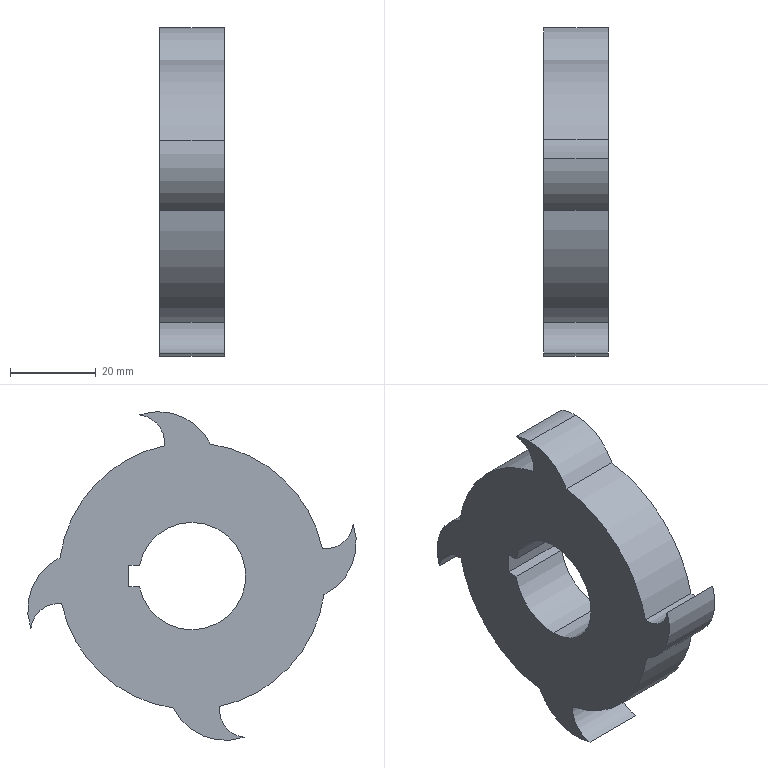Component | SolidWorks | CrushingCutterDisc-1 | 1 solid | 22 faces | box 15 x 76.47 x 76.47 mm | volume 41680 mm3 | cylinder 17 | plane 5 | commonest cylinder face diameters 12.958 x5 26.806 x5 62 x4 25 x3
build123d program:
from build123d import *

# Parameters (mm, degrees)
BOSS_EXTRUDE1_DEPTH = 15
CUT_EXTRUDE1_DEPTH  = 15


with BuildPart() as part:
    # Sketch1 → Boss-Extrude1 (new body)
    with BuildSketch(Plane.XY):
        with BuildLine():
            ThreePointArc((-30.696, -4.328), (-22.657, -21.158), (-6.415, -30.329))
            ThreePointArc((-6.415, -30.329), (-7.787, -35.094), (-12.127, -37.494))
            ThreePointArc((-12.127, -37.494), (-2.607, -37.222), (4.328, -30.696))
            ThreePointArc((4.328, -30.696), (21.158, -22.657), (30.329, -6.415))
            ThreePointArc((30.329, -6.415), (35.094, -7.787), (37.494, -12.127))
            ThreePointArc((37.494, -12.127), (37.222, -2.607), (30.696, 4.328))
            ThreePointArc((30.696, 4.328), (22.657, 21.158), (6.415, 30.329))
            ThreePointArc((6.415, 30.329), (7.787, 35.094), (12.127, 37.494))
            ThreePointArc((12.127, 37.494), (2.607, 37.222), (-4.328, 30.696))
            ThreePointArc((-4.328, 30.696), (-21.158, 22.657), (-30.329, 6.415))
            ThreePointArc((-30.329, 6.415), (-35.094, 7.787), (-37.494, 12.127))
            ThreePointArc((-37.494, 12.127), (-37.222, 2.607), (-30.696, -4.328))
        make_face()
    extrude(amount=BOSS_EXTRUDE1_DEPTH)

    # Sketch2 → Cut-Extrude1 (cut)
    with BuildSketch(Plane.XY.offset(15)):
        with BuildLine():
            Line((-2.499, 12.248), (-2.499, 14.709))
            Line((-2.499, 14.709), (2.501, 14.709))
            Line((2.501, 14.709), (2.501, 12.247))
            ThreePointArc((2.501, 12.247), (-0.001021, -12.5), (-2.499, 12.248))
        make_face()
    extrude(amount=-CUT_EXTRUDE1_DEPTH, mode=Mode.SUBTRACT)


solid = part.part

# Placed as in the assembly
solid = solid.moved(Location((386.19, 335.1, -35), (0, 90, 0)))
STEP:
#1=COLOUR_RGB('',0.7922,0.8196,0.9333);
#2=FILL_AREA_STYLE_COLOUR('',#1);
#3=FILL_AREA_STYLE('',(#2));
#4=SURFACE_STYLE_FILL_AREA(#3);
#5=SURFACE_SIDE_STYLE('',(#4));
#6=SURFACE_STYLE_USAGE(.BOTH.,#5);
#7=PRESENTATION_STYLE_ASSIGNMENT((#6));
#8=CARTESIAN_POINT('',(15.204,13.193,-0.8858));
#9=VERTEX_POINT('',#8);
#10=CARTESIAN_POINT('',(15.204,13.193,-1.87));
#11=VERTEX_POINT('',#10);
#12=CARTESIAN_POINT('',(15.204,13.193,-1.378));
#13=DIRECTION('',(1.,0.,-0.));
#14=DIRECTION('',(0.,0.,-1.));
#15=AXIS2_PLACEMENT_3D('',#12,#13,#14);
#16=CIRCLE('',#15,0.4921);
#17=EDGE_CURVE('',#9,#11,#16,.T.);
#18=ORIENTED_EDGE('',*,*,#17,.F.);
#19=CARTESIAN_POINT('',(15.795,13.193,-0.8858));
#20=VERTEX_POINT('',#19);
#21=CARTESIAN_POINT('',(15.204,13.193,-0.8858));
#22=DIRECTION('',(1.,0.,-0.));
#23=VECTOR('',#22,39.37);
#24=LINE('',#21,#23);
#25=EDGE_CURVE('',#9,#20,#24,.T.);
#26=ORIENTED_EDGE('',*,*,#25,.T.);
#27=CARTESIAN_POINT('',(15.795,13.193,-1.87));
#28=VERTEX_POINT('',#27);
#29=CARTESIAN_POINT('',(15.795,13.193,-1.378));
#30=DIRECTION('',(1.,0.,-0.));
#31=DIRECTION('',(0.,0.,-1.));
#32=AXIS2_PLACEMENT_3D('',#29,#30,#31);
#33=CIRCLE('',#32,0.4921);
#34=EDGE_CURVE('',#20,#28,#33,.T.);
#35=ORIENTED_EDGE('',*,*,#34,.T.);
#36=CARTESIAN_POINT('',(15.204,13.193,-1.87));
#37=DIRECTION('',(1.,0.,-0.));
#38=VECTOR('',#37,39.37);
#39=LINE('',#36,#38);
#40=EDGE_CURVE('',#11,#28,#39,.T.);
#41=ORIENTED_EDGE('',*,*,#40,.F.);
#42=EDGE_LOOP('',(#18,#26,#35,#41));
#43=FACE_OUTER_BOUND('',#42,.T.);
#44=CARTESIAN_POINT('',(15.204,13.193,-1.378));
#45=DIRECTION('',(1.,0.,-0.));
#46=DIRECTION('',(0.,0.,-1.));
#47=AXIS2_PLACEMENT_3D('',#44,#45,#46);
#48=CYLINDRICAL_SURFACE('',#47,0.4921);
#49=ADVANCED_FACE('',(#43),#48,.F.);
#50=CARTESIAN_POINT('',(15.204,13.675,-1.476));
#51=VERTEX_POINT('',#50);
#52=CARTESIAN_POINT('',(15.204,13.193,-1.378));
#53=DIRECTION('',(1.,0.,-0.));
#54=DIRECTION('',(0.,0.,-1.));
#55=AXIS2_PLACEMENT_3D('',#52,#53,#54);
#56=CIRCLE('',#55,0.4921);
#57=EDGE_CURVE('',#11,#51,#56,.T.);
#58=ORIENTED_EDGE('',*,*,#57,.F.);
#59=ORIENTED_EDGE('',*,*,#40,.T.);
#60=CARTESIAN_POINT('',(15.795,13.675,-1.476));
#61=VERTEX_POINT('',#60);
#62=CARTESIAN_POINT('',(15.795,13.193,-1.378));
#63=DIRECTION('',(1.,0.,-0.));
#64=DIRECTION('',(0.,0.,-1.));
#65=AXIS2_PLACEMENT_3D('',#62,#63,#64);
#66=CIRCLE('',#65,0.4921);
#67=EDGE_CURVE('',#28,#61,#66,.T.);
#68=ORIENTED_EDGE('',*,*,#67,.T.);
#69=CARTESIAN_POINT('',(15.204,13.675,-1.476));
#70=DIRECTION('',(1.,0.,-0.));
#71=VECTOR('',#70,39.37);
#72=LINE('',#69,#71);
#73=EDGE_CURVE('',#51,#61,#72,.T.);
#74=ORIENTED_EDGE('',*,*,#73,.F.);
#75=EDGE_LOOP('',(#58,#59,#68,#74));
#76=FACE_OUTER_BOUND('',#75,.T.);
#77=CARTESIAN_POINT('',(15.204,13.193,-1.378));
#78=DIRECTION('',(1.,0.,-0.));
#79=DIRECTION('',(0.,0.,-1.));
#80=AXIS2_PLACEMENT_3D('',#77,#78,#79);
#81=CYLINDRICAL_SURFACE('',#80,0.4921);
#82=ADVANCED_FACE('',(#76),#81,.F.);
#83=CARTESIAN_POINT('',(15.795,14.416,-1.629));
#84=VERTEX_POINT('',#83);
#85=CARTESIAN_POINT('',(15.795,14.669,-1.855));
#86=VERTEX_POINT('',#85);
#87=CARTESIAN_POINT('',(15.795,14.416,-1.884));
#88=DIRECTION('',(-1.,-0.,0.));
#89=DIRECTION('',(0.,0.,1.));
#90=AXIS2_PLACEMENT_3D('',#87,#88,#89);
#91=CIRCLE('',#90,0.2551);
#92=EDGE_CURVE('',#84,#86,#91,.T.);
#93=ORIENTED_EDGE('',*,*,#92,.F.);
#94=CARTESIAN_POINT('',(15.204,14.416,-1.629));
#95=VERTEX_POINT('',#94);
#96=CARTESIAN_POINT('',(15.795,14.416,-1.629));
#97=DIRECTION('',(-1.,-0.,0.));
#98=VECTOR('',#97,39.37);
#99=LINE('',#96,#98);
#100=EDGE_CURVE('',#84,#95,#99,.T.);
#101=ORIENTED_EDGE('',*,*,#100,.T.);
#102=CARTESIAN_POINT('',(15.204,14.669,-1.855));
#103=VERTEX_POINT('',#102);
#104=CARTESIAN_POINT('',(15.204,14.416,-1.884));
#105=DIRECTION('',(-1.,-0.,0.));
#106=DIRECTION('',(0.,0.,1.));
#107=AXIS2_PLACEMENT_3D('',#104,#105,#106);
#108=CIRCLE('',#107,0.2551);
#109=EDGE_CURVE('',#95,#103,#108,.T.);
#110=ORIENTED_EDGE('',*,*,#109,.T.);
#111=CARTESIAN_POINT('',(15.795,14.669,-1.855));
#112=DIRECTION('',(-1.,-0.,0.));
#113=VECTOR('',#112,39.37);
#114=LINE('',#111,#113);
#115=EDGE_CURVE('',#86,#103,#114,.T.);
#116=ORIENTED_EDGE('',*,*,#115,.F.);
#117=EDGE_LOOP('',(#93,#101,#110,#116));
#118=FACE_OUTER_BOUND('',#117,.T.);
#119=CARTESIAN_POINT('',(15.795,14.416,-1.884));
#120=DIRECTION('',(-1.,-0.,0.));
#121=DIRECTION('',(0.,0.,1.));
#122=AXIS2_PLACEMENT_3D('',#119,#120,#121);
#123=CYLINDRICAL_SURFACE('',#122,0.2551);
#124=ADVANCED_FACE('',(#118),#123,.F.);
#125=CARTESIAN_POINT('',(15.795,13.497,0.1275));
#126=VERTEX_POINT('',#125);
#127=CARTESIAN_POINT('',(15.795,13.023,-0.1694));
#128=VERTEX_POINT('',#127);
#129=CARTESIAN_POINT('',(15.795,13.497,-0.4002));
#130=DIRECTION('',(1.,0.,-0.));
#131=DIRECTION('',(0.,0.,1.));
#132=AXIS2_PLACEMENT_3D('',#129,#130,#131);
#133=CIRCLE('',#132,0.5277);
#134=EDGE_CURVE('',#126,#128,#133,.T.);
#135=ORIENTED_EDGE('',*,*,#134,.F.);
#136=CARTESIAN_POINT('',(15.204,13.497,0.1275));
#137=VERTEX_POINT('',#136);
#138=CARTESIAN_POINT('',(15.795,13.497,0.1275));
#139=DIRECTION('',(-1.,-0.,0.));
#140=VECTOR('',#139,39.37);
#141=LINE('',#138,#140);
#142=EDGE_CURVE('',#126,#137,#141,.T.);
#143=ORIENTED_EDGE('',*,*,#142,.T.);
#144=CARTESIAN_POINT('',(15.204,13.023,-0.1694));
#145=VERTEX_POINT('',#144);
#146=CARTESIAN_POINT('',(15.204,13.497,-0.4002));
#147=DIRECTION('',(1.,0.,-0.));
#148=DIRECTION('',(0.,0.,1.));
#149=AXIS2_PLACEMENT_3D('',#146,#147,#148);
#150=CIRCLE('',#149,0.5277);
#151=EDGE_CURVE('',#137,#145,#150,.T.);
#152=ORIENTED_EDGE('',*,*,#151,.T.);
#153=CARTESIAN_POINT('',(15.795,13.023,-0.1694));
#154=DIRECTION('',(-1.,-0.,0.));
#155=VECTOR('',#154,39.37);
#156=LINE('',#153,#155);
#157=EDGE_CURVE('',#128,#145,#156,.T.);
#158=ORIENTED_EDGE('',*,*,#157,.F.);
#159=EDGE_LOOP('',(#135,#143,#152,#158));
#160=FACE_OUTER_BOUND('',#159,.T.);
#161=CARTESIAN_POINT('',(15.795,13.497,-0.4002));
#162=DIRECTION('',(-1.,-0.,0.));
#163=DIRECTION('',(0.,0.,1.));
#164=AXIS2_PLACEMENT_3D('',#161,#162,#163);
#165=CYLINDRICAL_SURFACE('',#164,0.5277);
#166=ADVANCED_FACE('',(#160),#165,.T.);
#167=CARTESIAN_POINT('',(15.204,14.401,-1.208));
#168=VERTEX_POINT('',#167);
#169=CARTESIAN_POINT('',(15.204,13.445,-0.1839));
#170=VERTEX_POINT('',#169);
#171=CARTESIAN_POINT('',(15.204,13.193,-1.378));
#172=DIRECTION('',(1.,0.,-0.));
#173=DIRECTION('',(0.,0.,-1.));
#174=AXIS2_PLACEMENT_3D('',#171,#172,#173);
#175=CIRCLE('',#174,1.22);
#176=EDGE_CURVE('',#168,#170,#175,.T.);
#177=ORIENTED_EDGE('',*,*,#176,.T.);
#178=CARTESIAN_POINT('',(15.795,13.445,-0.1839));
#179=VERTEX_POINT('',#178);
#180=CARTESIAN_POINT('',(15.795,13.445,-0.1839));
#181=DIRECTION('',(-1.,-0.,0.));
#182=VECTOR('',#181,39.37);
#183=LINE('',#180,#182);
#184=EDGE_CURVE('',#179,#170,#183,.T.);
#185=ORIENTED_EDGE('',*,*,#184,.F.);
#186=CARTESIAN_POINT('',(15.795,14.401,-1.208));
#187=VERTEX_POINT('',#186);
#188=CARTESIAN_POINT('',(15.795,13.193,-1.378));
#189=DIRECTION('',(1.,0.,-0.));
#190=DIRECTION('',(0.,0.,-1.));
#191=AXIS2_PLACEMENT_3D('',#188,#189,#190);
#192=CIRCLE('',#191,1.22);
#193=EDGE_CURVE('',#187,#179,#192,.T.);
#194=ORIENTED_EDGE('',*,*,#193,.F.);
#195=CARTESIAN_POINT('',(15.795,14.401,-1.208));
#196=DIRECTION('',(-1.,-0.,0.));
#197=VECTOR('',#196,39.37);
#198=LINE('',#195,#197);
#199=EDGE_CURVE('',#187,#168,#198,.T.);
#200=ORIENTED_EDGE('',*,*,#199,.T.);
#201=EDGE_LOOP('',(#177,#185,#194,#200));
#202=FACE_OUTER_BOUND('',#201,.T.);
#203=CARTESIAN_POINT('',(15.795,13.193,-1.378));
#204=DIRECTION('',(-1.,-0.,0.));
#205=DIRECTION('',(0.,0.,1.));
#206=AXIS2_PLACEMENT_3D('',#203,#204,#205);
#207=CYLINDRICAL_SURFACE('',#206,1.22);
#208=ADVANCED_FACE('',(#202),#207,.T.);
#209=CARTESIAN_POINT('',(15.204,13.67,0.09819));
#210=VERTEX_POINT('',#209);
#211=CARTESIAN_POINT('',(15.204,13.699,-0.1553));
#212=DIRECTION('',(-1.,-0.,0.));
#213=DIRECTION('',(0.,0.,1.));
#214=AXIS2_PLACEMENT_3D('',#211,#212,#213);
#215=CIRCLE('',#214,0.2551);
#216=EDGE_CURVE('',#170,#210,#215,.T.);
#217=ORIENTED_EDGE('',*,*,#216,.T.);
#218=CARTESIAN_POINT('',(15.795,13.67,0.09819));
#219=VERTEX_POINT('',#218);
#220=CARTESIAN_POINT('',(15.795,13.67,0.09819));
#221=DIRECTION('',(-1.,-0.,0.));
#222=VECTOR('',#221,39.37);
#223=LINE('',#220,#222);
#224=EDGE_CURVE('',#219,#210,#223,.T.);
#225=ORIENTED_EDGE('',*,*,#224,.F.);
#226=CARTESIAN_POINT('',(15.795,13.699,-0.1553));
#227=DIRECTION('',(-1.,-0.,0.));
#228=DIRECTION('',(0.,0.,1.));
#229=AXIS2_PLACEMENT_3D('',#226,#227,#228);
#230=CIRCLE('',#229,0.2551);
#231=EDGE_CURVE('',#179,#219,#230,.T.);
#232=ORIENTED_EDGE('',*,*,#231,.F.);
#233=ORIENTED_EDGE('',*,*,#184,.T.);
#234=EDGE_LOOP('',(#217,#225,#232,#233));
#235=FACE_OUTER_BOUND('',#234,.T.);
#236=CARTESIAN_POINT('',(15.795,13.699,-0.1553));
#237=DIRECTION('',(-1.,-0.,0.));
#238=DIRECTION('',(0.,0.,1.));
#239=AXIS2_PLACEMENT_3D('',#236,#237,#238);
#240=CYLINDRICAL_SURFACE('',#239,0.2551);
#241=ADVANCED_FACE('',(#235),#240,.F.);
#242=ORIENTED_EDGE('',*,*,#142,.F.);
#243=CARTESIAN_POINT('',(15.795,13.497,-0.4002));
#244=DIRECTION('',(1.,0.,-0.));
#245=DIRECTION('',(0.,0.,1.));
#246=AXIS2_PLACEMENT_3D('',#243,#244,#245);
#247=CIRCLE('',#246,0.5277);
#248=EDGE_CURVE('',#219,#126,#247,.T.);
#249=ORIENTED_EDGE('',*,*,#248,.F.);
#250=ORIENTED_EDGE('',*,*,#224,.T.);
#251=CARTESIAN_POINT('',(15.204,13.497,-0.4002));
#252=DIRECTION('',(1.,0.,-0.));
#253=DIRECTION('',(0.,0.,1.));
#254=AXIS2_PLACEMENT_3D('',#251,#252,#253);
#255=CIRCLE('',#254,0.5277);
#256=EDGE_CURVE('',#210,#137,#255,.T.);
#257=ORIENTED_EDGE('',*,*,#256,.T.);
#258=EDGE_LOOP('',(#242,#249,#250,#257));
#259=FACE_OUTER_BOUND('',#258,.T.);
#260=CARTESIAN_POINT('',(15.795,13.497,-0.4002));
#261=DIRECTION('',(-1.,-0.,0.));
#262=DIRECTION('',(0.,0.,1.));
#263=AXIS2_PLACEMENT_3D('',#260,#261,#262);
#264=CYLINDRICAL_SURFACE('',#263,0.5277);
#265=ADVANCED_FACE('',(#259),#264,.T.);
#266=CARTESIAN_POINT('',(15.204,11.999,-1.125));
#267=VERTEX_POINT('',#266);
#268=CARTESIAN_POINT('',(15.204,13.193,-1.378));
#269=DIRECTION('',(1.,0.,-0.));
#270=DIRECTION('',(0.,0.,-1.));
#271=AXIS2_PLACEMENT_3D('',#268,#269,#270);
#272=CIRCLE('',#271,1.22);
#273=EDGE_CURVE('',#145,#267,#272,.T.);
#274=ORIENTED_EDGE('',*,*,#273,.T.);
#275=CARTESIAN_POINT('',(15.795,11.999,-1.125));
#276=VERTEX_POINT('',#275);
#277=CARTESIAN_POINT('',(15.795,11.999,-1.125));
#278=DIRECTION('',(-1.,-0.,0.));
#279=VECTOR('',#278,39.37);
#280=LINE('',#277,#279);
#281=EDGE_CURVE('',#276,#267,#280,.T.);
#282=ORIENTED_EDGE('',*,*,#281,.F.);
#283=CARTESIAN_POINT('',(15.795,13.193,-1.378));
#284=DIRECTION('',(1.,0.,-0.));
#285=DIRECTION('',(0.,0.,-1.));
#286=AXIS2_PLACEMENT_3D('',#283,#284,#285);
#287=CIRCLE('',#286,1.22);
#288=EDGE_CURVE('',#128,#276,#287,.T.);
#289=ORIENTED_EDGE('',*,*,#288,.F.);
#290=ORIENTED_EDGE('',*,*,#157,.T.);
#291=EDGE_LOOP('',(#274,#282,#289,#290));
#292=FACE_OUTER_BOUND('',#291,.T.);
#293=CARTESIAN_POINT('',(15.795,13.193,-1.378));
#294=DIRECTION('',(-1.,-0.,0.));
#295=DIRECTION('',(0.,0.,1.));
#296=AXIS2_PLACEMENT_3D('',#293,#294,#295);
#297=CYLINDRICAL_SURFACE('',#296,1.22);
#298=ADVANCED_FACE('',(#292),#297,.T.);
#299=CARTESIAN_POINT('',(15.204,11.717,-0.9005));
#300=VERTEX_POINT('',#299);
#301=CARTESIAN_POINT('',(15.204,11.97,-0.8719));
#302=DIRECTION('',(-1.,-0.,0.));
#303=DIRECTION('',(0.,0.,1.));
#304=AXIS2_PLACEMENT_3D('',#301,#302,#303);
#305=CIRCLE('',#304,0.2551);
#306=EDGE_CURVE('',#267,#300,#305,.T.);
#307=ORIENTED_EDGE('',*,*,#306,.T.);
#308=CARTESIAN_POINT('',(15.795,11.717,-0.9005));
#309=VERTEX_POINT('',#308);
#310=CARTESIAN_POINT('',(15.795,11.717,-0.9005));
#311=DIRECTION('',(-1.,-0.,0.));
#312=VECTOR('',#311,39.37);
#313=LINE('',#310,#312);
#314=EDGE_CURVE('',#309,#300,#313,.T.);
#315=ORIENTED_EDGE('',*,*,#314,.F.);
#316=CARTESIAN_POINT('',(15.795,11.97,-0.8719));
#317=DIRECTION('',(-1.,-0.,0.));
#318=DIRECTION('',(0.,0.,1.));
#319=AXIS2_PLACEMENT_3D('',#316,#317,#318);
#320=CIRCLE('',#319,0.2551);
#321=EDGE_CURVE('',#276,#309,#320,.T.);
#322=ORIENTED_EDGE('',*,*,#321,.F.);
#323=ORIENTED_EDGE('',*,*,#281,.T.);
#324=EDGE_LOOP('',(#307,#315,#322,#323));
#325=FACE_OUTER_BOUND('',#324,.T.);
#326=CARTESIAN_POINT('',(15.795,11.97,-0.8719));
#327=DIRECTION('',(-1.,-0.,0.));
#328=DIRECTION('',(0.,0.,1.));
#329=AXIS2_PLACEMENT_3D('',#326,#327,#328);
#330=CYLINDRICAL_SURFACE('',#329,0.2551);
#331=ADVANCED_FACE('',(#325),#330,.F.);
#332=CARTESIAN_POINT('',(15.204,11.984,-1.548));
#333=VERTEX_POINT('',#332);
#334=CARTESIAN_POINT('',(15.204,12.215,-1.074));
#335=DIRECTION('',(1.,0.,-0.));
#336=DIRECTION('',(0.,0.,1.));
#337=AXIS2_PLACEMENT_3D('',#334,#335,#336);
#338=CIRCLE('',#337,0.5277);
#339=EDGE_CURVE('',#300,#333,#338,.T.);
#340=ORIENTED_EDGE('',*,*,#339,.T.);
#341=CARTESIAN_POINT('',(15.795,11.984,-1.548));
#342=VERTEX_POINT('',#341);
#343=CARTESIAN_POINT('',(15.795,11.984,-1.548));
#344=DIRECTION('',(-1.,-0.,0.));
#345=VECTOR('',#344,39.37);
#346=LINE('',#343,#345);
#347=EDGE_CURVE('',#342,#333,#346,.T.);
#348=ORIENTED_EDGE('',*,*,#347,.F.);
#349=CARTESIAN_POINT('',(15.795,12.215,-1.074));
#350=DIRECTION('',(1.,0.,-0.));
#351=DIRECTION('',(0.,0.,1.));
#352=AXIS2_PLACEMENT_3D('',#349,#350,#351);
#353=CIRCLE('',#352,0.5277);
#354=EDGE_CURVE('',#309,#342,#353,.T.);
#355=ORIENTED_EDGE('',*,*,#354,.F.);
#356=ORIENTED_EDGE('',*,*,#314,.T.);
#357=EDGE_LOOP('',(#340,#348,#355,#356));
#358=FACE_OUTER_BOUND('',#357,.T.);
#359=CARTESIAN_POINT('',(15.795,12.215,-1.074));
#360=DIRECTION('',(-1.,-0.,0.));
#361=DIRECTION('',(0.,0.,1.));
#362=AXIS2_PLACEMENT_3D('',#359,#360,#361);
#363=CYLINDRICAL_SURFACE('',#362,0.5277);
#364=ADVANCED_FACE('',(#358),#363,.T.);
#365=CARTESIAN_POINT('',(15.204,12.94,-2.572));
#366=VERTEX_POINT('',#365);
#367=CARTESIAN_POINT('',(15.204,13.193,-1.378));
#368=DIRECTION('',(1.,0.,-0.));
#369=DIRECTION('',(0.,0.,-1.));
#370=AXIS2_PLACEMENT_3D('',#367,#368,#369);
#371=CIRCLE('',#370,1.22);
#372=EDGE_CURVE('',#333,#366,#371,.T.);
#373=ORIENTED_EDGE('',*,*,#372,.T.);
#374=CARTESIAN_POINT('',(15.795,12.94,-2.572));
#375=VERTEX_POINT('',#374);
#376=CARTESIAN_POINT('',(15.795,12.94,-2.572));
#377=DIRECTION('',(-1.,-0.,0.));
#378=VECTOR('',#377,39.37);
#379=LINE('',#376,#378);
#380=EDGE_CURVE('',#375,#366,#379,.T.);
#381=ORIENTED_EDGE('',*,*,#380,.F.);
#382=CARTESIAN_POINT('',(15.795,13.193,-1.378));
#383=DIRECTION('',(1.,0.,-0.));
#384=DIRECTION('',(0.,0.,-1.));
#385=AXIS2_PLACEMENT_3D('',#382,#383,#384);
#386=CIRCLE('',#385,1.22);
#387=EDGE_CURVE('',#342,#375,#386,.T.);
#388=ORIENTED_EDGE('',*,*,#387,.F.);
#389=ORIENTED_EDGE('',*,*,#347,.T.);
#390=EDGE_LOOP('',(#373,#381,#388,#389));
#391=FACE_OUTER_BOUND('',#390,.T.);
#392=CARTESIAN_POINT('',(15.795,13.193,-1.378));
#393=DIRECTION('',(-1.,-0.,0.));
#394=DIRECTION('',(0.,0.,1.));
#395=AXIS2_PLACEMENT_3D('',#392,#393,#394);
#396=CYLINDRICAL_SURFACE('',#395,1.22);
#397=ADVANCED_FACE('',(#391),#396,.T.);
#398=CARTESIAN_POINT('',(15.204,12.715,-2.854));
#399=VERTEX_POINT('',#398);
#400=CARTESIAN_POINT('',(15.204,12.687,-2.601));
#401=DIRECTION('',(-1.,-0.,0.));
#402=DIRECTION('',(0.,0.,1.));
#403=AXIS2_PLACEMENT_3D('',#400,#401,#402);
#404=CIRCLE('',#403,0.2551);
#405=EDGE_CURVE('',#366,#399,#404,.T.);
#406=ORIENTED_EDGE('',*,*,#405,.T.);
#407=CARTESIAN_POINT('',(15.795,12.715,-2.854));
#408=VERTEX_POINT('',#407);
#409=CARTESIAN_POINT('',(15.795,12.715,-2.854));
#410=DIRECTION('',(-1.,-0.,0.));
#411=VECTOR('',#410,39.37);
#412=LINE('',#409,#411);
#413=EDGE_CURVE('',#408,#399,#412,.T.);
#414=ORIENTED_EDGE('',*,*,#413,.F.);
#415=CARTESIAN_POINT('',(15.795,12.687,-2.601));
#416=DIRECTION('',(-1.,-0.,0.));
#417=DIRECTION('',(0.,0.,1.));
#418=AXIS2_PLACEMENT_3D('',#415,#416,#417);
#419=CIRCLE('',#418,0.2551);
#420=EDGE_CURVE('',#375,#408,#419,.T.);
#421=ORIENTED_EDGE('',*,*,#420,.F.);
#422=ORIENTED_EDGE('',*,*,#380,.T.);
#423=EDGE_LOOP('',(#406,#414,#421,#422));
#424=FACE_OUTER_BOUND('',#423,.T.);
#425=CARTESIAN_POINT('',(15.795,12.687,-2.601));
#426=DIRECTION('',(-1.,-0.,0.));
#427=DIRECTION('',(0.,0.,1.));
#428=AXIS2_PLACEMENT_3D('',#425,#426,#427);
#429=CYLINDRICAL_SURFACE('',#428,0.2551);
#430=ADVANCED_FACE('',(#424),#429,.F.);
#431=CARTESIAN_POINT('',(15.204,13.363,-2.586));
#432=VERTEX_POINT('',#431);
#433=CARTESIAN_POINT('',(15.204,12.889,-2.356));
#434=DIRECTION('',(1.,0.,-0.));
#435=DIRECTION('',(0.,0.,1.));
#436=AXIS2_PLACEMENT_3D('',#433,#434,#435);
#437=CIRCLE('',#436,0.5277);
#438=EDGE_CURVE('',#399,#432,#437,.T.);
#439=ORIENTED_EDGE('',*,*,#438,.T.);
#440=CARTESIAN_POINT('',(15.795,13.363,-2.586));
#441=VERTEX_POINT('',#440);
#442=CARTESIAN_POINT('',(15.795,13.363,-2.586));
#443=DIRECTION('',(-1.,-0.,0.));
#444=VECTOR('',#443,39.37);
#445=LINE('',#442,#444);
#446=EDGE_CURVE('',#441,#432,#445,.T.);
#447=ORIENTED_EDGE('',*,*,#446,.F.);
#448=CARTESIAN_POINT('',(15.795,12.889,-2.356));
#449=DIRECTION('',(1.,0.,-0.));
#450=DIRECTION('',(0.,0.,1.));
#451=AXIS2_PLACEMENT_3D('',#448,#449,#450);
#452=CIRCLE('',#451,0.5277);
#453=EDGE_CURVE('',#408,#441,#452,.T.);
#454=ORIENTED_EDGE('',*,*,#453,.F.);
#455=ORIENTED_EDGE('',*,*,#413,.T.);
#456=EDGE_LOOP('',(#439,#447,#454,#455));
#457=FACE_OUTER_BOUND('',#456,.T.);
#458=CARTESIAN_POINT('',(15.795,12.889,-2.356));
#459=DIRECTION('',(-1.,-0.,0.));
#460=DIRECTION('',(0.,0.,1.));
#461=AXIS2_PLACEMENT_3D('',#458,#459,#460);
#462=CYLINDRICAL_SURFACE('',#461,0.5277);
#463=ADVANCED_FACE('',(#457),#462,.T.);
#464=CARTESIAN_POINT('',(15.204,14.387,-1.631));
#465=VERTEX_POINT('',#464);
#466=CARTESIAN_POINT('',(15.204,13.193,-1.378));
#467=DIRECTION('',(1.,0.,-0.));
#468=DIRECTION('',(0.,0.,-1.));
#469=AXIS2_PLACEMENT_3D('',#466,#467,#468);
#470=CIRCLE('',#469,1.22);
#471=EDGE_CURVE('',#432,#465,#470,.T.);
#472=ORIENTED_EDGE('',*,*,#471,.T.);
#473=CARTESIAN_POINT('',(15.795,14.387,-1.631));
#474=VERTEX_POINT('',#473);
#475=CARTESIAN_POINT('',(15.795,14.387,-1.631));
#476=DIRECTION('',(-1.,-0.,0.));
#477=VECTOR('',#476,39.37);
#478=LINE('',#475,#477);
#479=EDGE_CURVE('',#474,#465,#478,.T.);
#480=ORIENTED_EDGE('',*,*,#479,.F.);
#481=CARTESIAN_POINT('',(15.795,13.193,-1.378));
#482=DIRECTION('',(1.,0.,-0.));
#483=DIRECTION('',(0.,0.,-1.));
#484=AXIS2_PLACEMENT_3D('',#481,#482,#483);
#485=CIRCLE('',#484,1.22);
#486=EDGE_CURVE('',#441,#474,#485,.T.);
#487=ORIENTED_EDGE('',*,*,#486,.F.);
#488=ORIENTED_EDGE('',*,*,#446,.T.);
#489=EDGE_LOOP('',(#472,#480,#487,#488));
#490=FACE_OUTER_BOUND('',#489,.T.);
#491=CARTESIAN_POINT('',(15.795,13.193,-1.378));
#492=DIRECTION('',(-1.,-0.,0.));
#493=DIRECTION('',(0.,0.,1.));
#494=AXIS2_PLACEMENT_3D('',#491,#492,#493);
#495=CYLINDRICAL_SURFACE('',#494,1.22);
#496=ADVANCED_FACE('',(#490),#495,.T.);
#497=ORIENTED_EDGE('',*,*,#100,.F.);
#498=CARTESIAN_POINT('',(15.795,14.416,-1.884));
#499=DIRECTION('',(-1.,-0.,0.));
#500=DIRECTION('',(0.,0.,1.));
#501=AXIS2_PLACEMENT_3D('',#498,#499,#500);
#502=CIRCLE('',#501,0.2551);
#503=EDGE_CURVE('',#474,#84,#502,.T.);
#504=ORIENTED_EDGE('',*,*,#503,.F.);
#505=ORIENTED_EDGE('',*,*,#479,.T.);
#506=CARTESIAN_POINT('',(15.204,14.416,-1.884));
#507=DIRECTION('',(-1.,-0.,0.));
#508=DIRECTION('',(0.,0.,1.));
#509=AXIS2_PLACEMENT_3D('',#506,#507,#508);
#510=CIRCLE('',#509,0.2551);
#511=EDGE_CURVE('',#465,#95,#510,.T.);
#512=ORIENTED_EDGE('',*,*,#511,.T.);
#513=EDGE_LOOP('',(#497,#504,#505,#512));
#514=FACE_OUTER_BOUND('',#513,.T.);
#515=CARTESIAN_POINT('',(15.795,14.416,-1.884));
#516=DIRECTION('',(-1.,-0.,0.));
#517=DIRECTION('',(0.,0.,1.));
#518=AXIS2_PLACEMENT_3D('',#515,#516,#517);
#519=CYLINDRICAL_SURFACE('',#518,0.2551);
#520=ADVANCED_FACE('',(#514),#519,.F.);
#521=CARTESIAN_POINT('',(15.204,14.171,-1.682));
#522=DIRECTION('',(1.,0.,-0.));
#523=DIRECTION('',(0.,0.,1.));
#524=AXIS2_PLACEMENT_3D('',#521,#522,#523);
#525=CIRCLE('',#524,0.5277);
#526=EDGE_CURVE('',#103,#168,#525,.T.);
#527=ORIENTED_EDGE('',*,*,#526,.T.);
#528=ORIENTED_EDGE('',*,*,#199,.F.);
#529=CARTESIAN_POINT('',(15.795,14.171,-1.682));
#530=DIRECTION('',(1.,0.,-0.));
#531=DIRECTION('',(0.,0.,1.));
#532=AXIS2_PLACEMENT_3D('',#529,#530,#531);
#533=CIRCLE('',#532,0.5277);
#534=EDGE_CURVE('',#86,#187,#533,.T.);
#535=ORIENTED_EDGE('',*,*,#534,.F.);
#536=ORIENTED_EDGE('',*,*,#115,.T.);
#537=EDGE_LOOP('',(#527,#528,#535,#536));
#538=FACE_OUTER_BOUND('',#537,.T.);
#539=CARTESIAN_POINT('',(15.795,14.171,-1.682));
#540=DIRECTION('',(-1.,-0.,0.));
#541=DIRECTION('',(0.,0.,1.));
#542=AXIS2_PLACEMENT_3D('',#539,#540,#541);
#543=CYLINDRICAL_SURFACE('',#542,0.5277);
#544=ADVANCED_FACE('',(#538),#543,.T.);
#545=CARTESIAN_POINT('',(15.795,13.675,-1.28));
#546=VERTEX_POINT('',#545);
#547=CARTESIAN_POINT('',(15.795,13.193,-1.378));
#548=DIRECTION('',(1.,0.,-0.));
#549=DIRECTION('',(0.,0.,-1.));
#550=AXIS2_PLACEMENT_3D('',#547,#548,#549);
#551=CIRCLE('',#550,0.4921);
#552=EDGE_CURVE('',#546,#20,#551,.T.);
#553=ORIENTED_EDGE('',*,*,#552,.F.);
#554=CARTESIAN_POINT('',(15.795,13.772,-1.28));
#555=VERTEX_POINT('',#554);
#556=CARTESIAN_POINT('',(15.795,13.675,-1.28));
#557=DIRECTION('',(0.,-1.,-0.));
#558=VECTOR('',#557,39.37);
#559=LINE('',#556,#558);
#560=EDGE_CURVE('',#555,#546,#559,.T.);
#561=ORIENTED_EDGE('',*,*,#560,.F.);
#562=CARTESIAN_POINT('',(15.795,13.772,-1.476));
#563=VERTEX_POINT('',#562);
#564=CARTESIAN_POINT('',(15.795,13.772,-1.28));
#565=DIRECTION('',(0.,0.,1.));
#566=VECTOR('',#565,39.37);
#567=LINE('',#564,#566);
#568=EDGE_CURVE('',#563,#555,#567,.T.);
#569=ORIENTED_EDGE('',*,*,#568,.F.);
#570=CARTESIAN_POINT('',(15.795,13.772,-1.476));
#571=DIRECTION('',(-0.,1.,0.));
#572=VECTOR('',#571,39.37);
#573=LINE('',#570,#572);
#574=EDGE_CURVE('',#61,#563,#573,.T.);
#575=ORIENTED_EDGE('',*,*,#574,.F.);
#576=ORIENTED_EDGE('',*,*,#67,.F.);
#577=ORIENTED_EDGE('',*,*,#34,.F.);
#578=EDGE_LOOP('',(#553,#561,#569,#575,#576,#577));
#579=FACE_BOUND('',#578,.T.);
#580=ORIENTED_EDGE('',*,*,#193,.T.);
#581=ORIENTED_EDGE('',*,*,#231,.T.);
#582=ORIENTED_EDGE('',*,*,#248,.T.);
#583=ORIENTED_EDGE('',*,*,#134,.T.);
#584=ORIENTED_EDGE('',*,*,#288,.T.);
#585=ORIENTED_EDGE('',*,*,#321,.T.);
#586=ORIENTED_EDGE('',*,*,#354,.T.);
#587=ORIENTED_EDGE('',*,*,#387,.T.);
#588=ORIENTED_EDGE('',*,*,#420,.T.);
#589=ORIENTED_EDGE('',*,*,#453,.T.);
#590=ORIENTED_EDGE('',*,*,#486,.T.);
#591=ORIENTED_EDGE('',*,*,#503,.T.);
#592=ORIENTED_EDGE('',*,*,#92,.T.);
#593=ORIENTED_EDGE('',*,*,#534,.T.);
#594=EDGE_LOOP('',(#580,#581,#582,#583,#584,#585,#586,#587,#588,#589,#590,#591,#592,#593));
#595=FACE_OUTER_BOUND('',#594,.T.);
#596=CARTESIAN_POINT('',(15.795,13.446,-0.7666));
#597=DIRECTION('',(1.,0.,-0.));
#598=DIRECTION('',(-0.,0.,-1.));
#599=AXIS2_PLACEMENT_3D('',#596,#597,#598);
#600=PLANE('',#599);
#601=ADVANCED_FACE('',(#579,#595),#600,.T.);
#602=CARTESIAN_POINT('',(15.204,13.772,-1.28));
#603=VERTEX_POINT('',#602);
#604=CARTESIAN_POINT('',(15.204,13.675,-1.28));
#605=VERTEX_POINT('',#604);
#606=CARTESIAN_POINT('',(15.204,13.675,-1.28));
#607=DIRECTION('',(0.,-1.,-0.));
#608=VECTOR('',#607,39.37);
#609=LINE('',#606,#608);
#610=EDGE_CURVE('',#603,#605,#609,.T.);
#611=ORIENTED_EDGE('',*,*,#610,.T.);
#612=CARTESIAN_POINT('',(15.204,13.193,-1.378));
#613=DIRECTION('',(1.,0.,-0.));
#614=DIRECTION('',(0.,0.,-1.));
#615=AXIS2_PLACEMENT_3D('',#612,#613,#614);
#616=CIRCLE('',#615,0.4921);
#617=EDGE_CURVE('',#605,#9,#616,.T.);
#618=ORIENTED_EDGE('',*,*,#617,.T.);
#619=ORIENTED_EDGE('',*,*,#17,.T.);
#620=ORIENTED_EDGE('',*,*,#57,.T.);
#621=CARTESIAN_POINT('',(15.204,13.772,-1.476));
#622=VERTEX_POINT('',#621);
#623=CARTESIAN_POINT('',(15.204,13.772,-1.476));
#624=DIRECTION('',(-0.,1.,0.));
#625=VECTOR('',#624,39.37);
#626=LINE('',#623,#625);
#627=EDGE_CURVE('',#51,#622,#626,.T.);
#628=ORIENTED_EDGE('',*,*,#627,.T.);
#629=CARTESIAN_POINT('',(15.204,13.772,-1.28));
#630=DIRECTION('',(0.,0.,1.));
#631=VECTOR('',#630,39.37);
#632=LINE('',#629,#631);
#633=EDGE_CURVE('',#622,#603,#632,.T.);
#634=ORIENTED_EDGE('',*,*,#633,.T.);
#635=EDGE_LOOP('',(#611,#618,#619,#620,#628,#634));
#636=FACE_BOUND('',#635,.T.);
#637=ORIENTED_EDGE('',*,*,#176,.F.);
#638=ORIENTED_EDGE('',*,*,#526,.F.);
#639=ORIENTED_EDGE('',*,*,#109,.F.);
#640=ORIENTED_EDGE('',*,*,#511,.F.);
#641=ORIENTED_EDGE('',*,*,#471,.F.);
#642=ORIENTED_EDGE('',*,*,#438,.F.);
#643=ORIENTED_EDGE('',*,*,#405,.F.);
#644=ORIENTED_EDGE('',*,*,#372,.F.);
#645=ORIENTED_EDGE('',*,*,#339,.F.);
#646=ORIENTED_EDGE('',*,*,#306,.F.);
#647=ORIENTED_EDGE('',*,*,#273,.F.);
#648=ORIENTED_EDGE('',*,*,#151,.F.);
#649=ORIENTED_EDGE('',*,*,#256,.F.);
#650=ORIENTED_EDGE('',*,*,#216,.F.);
#651=EDGE_LOOP('',(#637,#638,#639,#640,#641,#642,#643,#644,#645,#646,#647,#648,#649,#650));
#652=FACE_OUTER_BOUND('',#651,.T.);
#653=CARTESIAN_POINT('',(15.204,13.446,-0.7666));
#654=DIRECTION('',(1.,0.,-0.));
#655=DIRECTION('',(-0.,0.,-1.));
#656=AXIS2_PLACEMENT_3D('',#653,#654,#655);
#657=PLANE('',#656);
#658=ADVANCED_FACE('',(#636,#652),#657,.F.);
#659=ORIENTED_EDGE('',*,*,#25,.F.);
#660=ORIENTED_EDGE('',*,*,#617,.F.);
#661=CARTESIAN_POINT('',(15.204,13.675,-1.28));
#662=DIRECTION('',(1.,0.,-0.));
#663=VECTOR('',#662,39.37);
#664=LINE('',#661,#663);
#665=EDGE_CURVE('',#605,#546,#664,.T.);
#666=ORIENTED_EDGE('',*,*,#665,.T.);
#667=ORIENTED_EDGE('',*,*,#552,.T.);
#668=EDGE_LOOP('',(#659,#660,#666,#667));
#669=FACE_OUTER_BOUND('',#668,.T.);
#670=CARTESIAN_POINT('',(15.204,13.193,-1.378));
#671=DIRECTION('',(1.,0.,-0.));
#672=DIRECTION('',(0.,0.,-1.));
#673=AXIS2_PLACEMENT_3D('',#670,#671,#672);
#674=CYLINDRICAL_SURFACE('',#673,0.4921);
#675=ADVANCED_FACE('',(#669),#674,.F.);
#676=ORIENTED_EDGE('',*,*,#560,.T.);
#677=ORIENTED_EDGE('',*,*,#665,.F.);
#678=ORIENTED_EDGE('',*,*,#610,.F.);
#679=CARTESIAN_POINT('',(15.204,13.772,-1.28));
#680=DIRECTION('',(1.,0.,-0.));
#681=VECTOR('',#680,39.37);
#682=LINE('',#679,#681);
#683=EDGE_CURVE('',#603,#555,#682,.T.);
#684=ORIENTED_EDGE('',*,*,#683,.T.);
#685=EDGE_LOOP('',(#676,#677,#678,#684));
#686=FACE_OUTER_BOUND('',#685,.T.);
#687=CARTESIAN_POINT('',(15.204,13.675,-1.28));
#688=DIRECTION('',(0.,0.,1.));
#689=DIRECTION('',(1.,0.,-0.));
#690=AXIS2_PLACEMENT_3D('',#687,#688,#689);
#691=PLANE('',#690);
#692=ADVANCED_FACE('',(#686),#691,.F.);
#693=ORIENTED_EDGE('',*,*,#568,.T.);
#694=ORIENTED_EDGE('',*,*,#683,.F.);
#695=ORIENTED_EDGE('',*,*,#633,.F.);
#696=CARTESIAN_POINT('',(15.204,13.772,-1.476));
#697=DIRECTION('',(1.,0.,-0.));
#698=VECTOR('',#697,39.37);
#699=LINE('',#696,#698);
#700=EDGE_CURVE('',#622,#563,#699,.T.);
#701=ORIENTED_EDGE('',*,*,#700,.T.);
#702=EDGE_LOOP('',(#693,#694,#695,#701));
#703=FACE_OUTER_BOUND('',#702,.T.);
#704=CARTESIAN_POINT('',(15.204,13.772,-1.28));
#705=DIRECTION('',(-0.,1.,-0.));
#706=DIRECTION('',(0.,0.,1.));
#707=AXIS2_PLACEMENT_3D('',#704,#705,#706);
#708=PLANE('',#707);
#709=ADVANCED_FACE('',(#703),#708,.F.);
#710=ORIENTED_EDGE('',*,*,#574,.T.);
#711=ORIENTED_EDGE('',*,*,#700,.F.);
#712=ORIENTED_EDGE('',*,*,#627,.F.);
#713=ORIENTED_EDGE('',*,*,#73,.T.);
#714=EDGE_LOOP('',(#710,#711,#712,#713));
#715=FACE_OUTER_BOUND('',#714,.T.);
#716=CARTESIAN_POINT('',(15.204,13.772,-1.476));
#717=DIRECTION('',(-0.,0.,-1.));
#718=DIRECTION('',(-0.,1.,0.));
#719=AXIS2_PLACEMENT_3D('',#716,#717,#718);
#720=PLANE('',#719);
#721=ADVANCED_FACE('',(#715),#720,.F.);
#722=CLOSED_SHELL('',(#49,#82,#124,#166,#208,#241,#265,#298,#331,#364,#397,#430,#463,#496,#520,#544,#601,#658,#675,#692,#709,#721));
#723=MANIFOLD_SOLID_BREP('',#722);
#724=STYLED_ITEM('',(#7),#723);
#725=(LENGTH_UNIT()NAMED_UNIT(*)SI_UNIT($,.METRE.));
#726=LENGTH_MEASURE_WITH_UNIT(LENGTH_MEASURE(0.0254),#725);
#727=DIMENSIONAL_EXPONENTS(1.,0.,0.,0.,0.,0.,0.);
#728=(CONVERSION_BASED_UNIT('',#726)LENGTH_UNIT()NAMED_UNIT(#727));
#729=UNCERTAINTY_MEASURE_WITH_UNIT(LENGTH_MEASURE(0.00001),#728,'','');
#730=(NAMED_UNIT(*)PLANE_ANGLE_UNIT()SI_UNIT($,.RADIAN.));
#731=(NAMED_UNIT(*)SI_UNIT($,.STERADIAN.)SOLID_ANGLE_UNIT());
#732=(GEOMETRIC_REPRESENTATION_CONTEXT(3)GLOBAL_UNCERTAINTY_ASSIGNED_CONTEXT((#729))GLOBAL_UNIT_ASSIGNED_CONTEXT((#728,#730,#731))REPRESENTATION_CONTEXT('',''));
#733=MECHANICAL_DESIGN_GEOMETRIC_PRESENTATION_REPRESENTATION('',(#724),#732);
#734=PRESENTATION_LAYER_ASSIGNMENT('','',(#724));
#735=CARTESIAN_POINT('',(0.,0.,0.));
#736=DIRECTION('',(0.,0.,1.));
#737=DIRECTION('',(1.,0.,0.));
#738=AXIS2_PLACEMENT_3D('',#735,#736,#737);
#739=(LENGTH_UNIT()NAMED_UNIT(*)SI_UNIT($,.METRE.));
#740=LENGTH_MEASURE_WITH_UNIT(LENGTH_MEASURE(0.0254),#739);
#741=DIMENSIONAL_EXPONENTS(1.,0.,0.,0.,0.,0.,0.);
#742=(CONVERSION_BASED_UNIT('',#740)LENGTH_UNIT()NAMED_UNIT(#741));
#743=UNCERTAINTY_MEASURE_WITH_UNIT(LENGTH_MEASURE(0.00001),#742,'','');
#744=(NAMED_UNIT(*)PLANE_ANGLE_UNIT()SI_UNIT($,.RADIAN.));
#745=(NAMED_UNIT(*)SI_UNIT($,.STERADIAN.)SOLID_ANGLE_UNIT());
#746=(GEOMETRIC_REPRESENTATION_CONTEXT(3)GLOBAL_UNCERTAINTY_ASSIGNED_CONTEXT((#743))GLOBAL_UNIT_ASSIGNED_CONTEXT((#742,#744,#745))REPRESENTATION_CONTEXT('',''));
#747=ADVANCED_BREP_SHAPE_REPRESENTATION('',(#723,#738),#746);